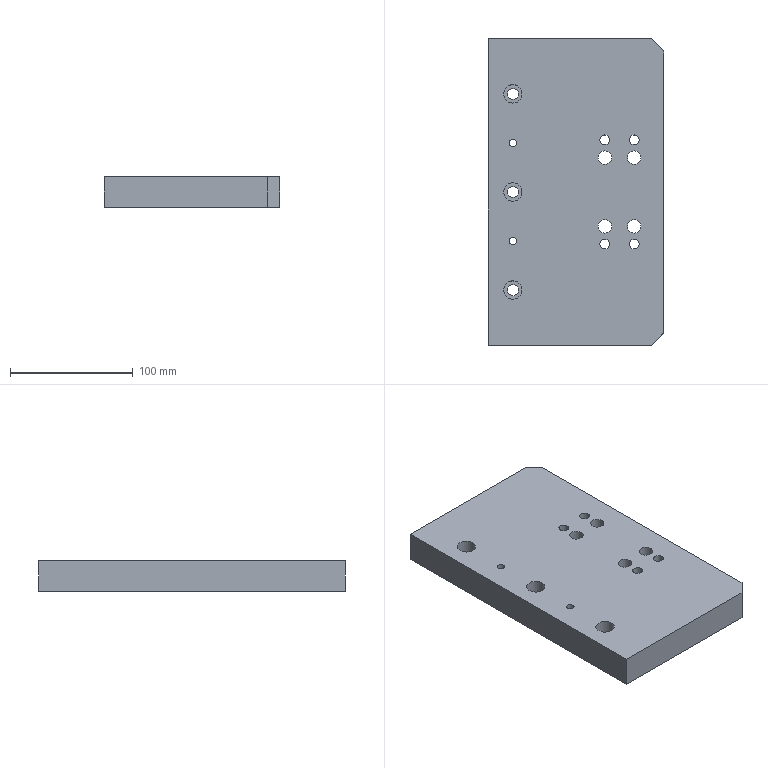Component | NX | SUPPORT_PLATE | 1 solid | 27 faces | volume 865446 mm3 | cylinder 16 | plane 11 | commonest cylinder face diameters 11 x4 8 x4 9 x3 15 x3 6 x2